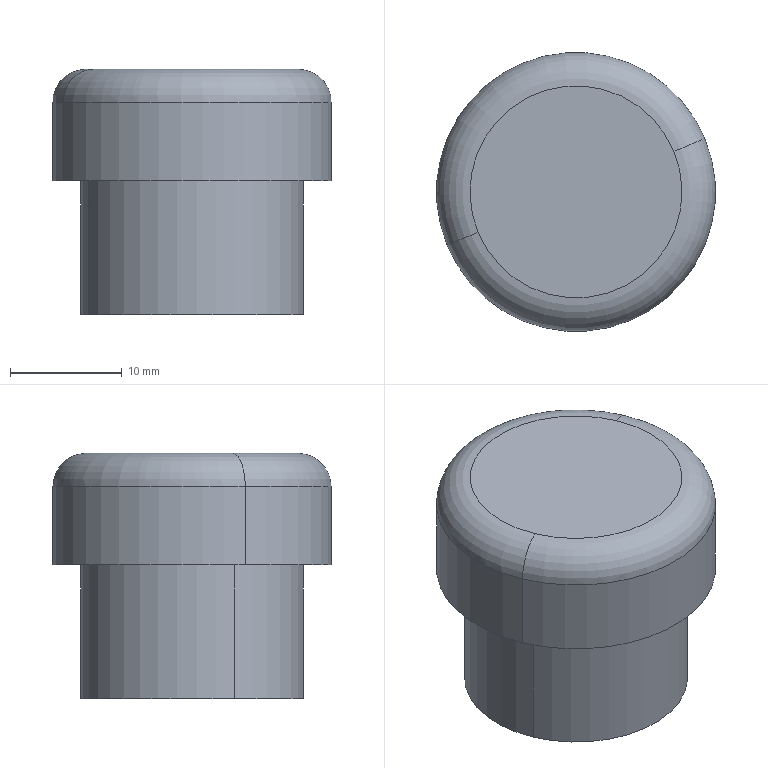Component | SolidWorks | DoubleFilmTransport-1_RubberPad-1 | 1 solid | 9 faces | box 25 x 25 x 22 mm | volume 8535 mm3 | cylinder 4 | plane 3 | torus 2 | commonest cylinder face diameters 25 x2 20 x2
build123d program:
from build123d import *


with BuildPart() as part:
    # Sketch1 → Revolve1 (revolve)
    with BuildSketch(Plane(origin=(0, 0, 0), x_dir=(-1, 0, 0), z_dir=(0, 0, -1)), mode=Mode.PRIVATE) as revolve1_sk:
        with BuildLine():
            Line((0, 10), (0, 0))
            Line((0, 0), (22, 0))
            Line((22, 0), (22, 9.5))
            ThreePointArc((22, 9.5), (21.121, 11.621), (19, 12.5))
            Line((19, 12.5), (12, 12.5))
            Line((12, 12.5), (12, 10))
            Line((12, 10), (0, 10))
        make_face()
    revolve(revolve1_sk.sketch.rotate(Axis((0, 0, 0), (-1, 0, 0)), 180), axis=Axis((0, 0, 0), (-1, 0, 0)))


solid = part.part

# Placed as in the assembly
solid = solid.moved(Location((-298.746, 95.373, 58.5), (0, 90, 0)))
STEP:
#1=CARTESIAN_POINT('',(-11.307,3.943,2.776));
#2=VERTEX_POINT('',#1);
#3=CARTESIAN_POINT('',(-12.217,3.567,2.776));
#4=VERTEX_POINT('',#3);
#5=CARTESIAN_POINT('',(-11.762,3.755,2.776));
#6=DIRECTION('',(0.,0.,1.));
#7=DIRECTION('',(0.9242,0.3818,0.));
#8=AXIS2_PLACEMENT_3D('',#5,#6,#7);
#9=CIRCLE('',#8,0.4921);
#10=EDGE_CURVE('',#2,#4,#9,.T.);
#11=ORIENTED_EDGE('',*,*,#10,.T.);
#12=CARTESIAN_POINT('',(-12.217,3.567,3.051));
#13=VERTEX_POINT('',#12);
#14=CARTESIAN_POINT('',(-12.217,3.567,2.303));
#15=DIRECTION('',(0.,0.,1.));
#16=VECTOR('',#15,39.37);
#17=LINE('',#14,#16);
#18=EDGE_CURVE('',#4,#13,#17,.T.);
#19=ORIENTED_EDGE('',*,*,#18,.T.);
#20=CARTESIAN_POINT('',(-11.307,3.943,3.051));
#21=VERTEX_POINT('',#20);
#22=CARTESIAN_POINT('',(-11.762,3.755,3.051));
#23=DIRECTION('',(0.,0.,1.));
#24=DIRECTION('',(0.9242,0.3818,0.));
#25=AXIS2_PLACEMENT_3D('',#22,#23,#24);
#26=CIRCLE('',#25,0.4921);
#27=EDGE_CURVE('',#21,#13,#26,.T.);
#28=ORIENTED_EDGE('',*,*,#27,.F.);
#29=CARTESIAN_POINT('',(-11.307,3.943,2.303));
#30=DIRECTION('',(0.,0.,1.));
#31=VECTOR('',#30,39.37);
#32=LINE('',#29,#31);
#33=EDGE_CURVE('',#2,#21,#32,.T.);
#34=ORIENTED_EDGE('',*,*,#33,.F.);
#35=EDGE_LOOP('',(#11,#19,#28,#34));
#36=FACE_OUTER_BOUND('',#35,.T.);
#37=CARTESIAN_POINT('',(-11.762,3.755,2.303));
#38=DIRECTION('',(0.,0.,1.));
#39=DIRECTION('',(0.9242,0.3818,0.));
#40=AXIS2_PLACEMENT_3D('',#37,#38,#39);
#41=CYLINDRICAL_SURFACE('',#40,0.4921);
#42=ADVANCED_FACE('',(#36),#41,.T.);
#43=ORIENTED_EDGE('',*,*,#27,.T.);
#44=CARTESIAN_POINT('',(-12.107,3.612,3.169));
#45=VERTEX_POINT('',#44);
#46=CARTESIAN_POINT('',(-12.107,3.612,3.051));
#47=DIRECTION('',(-0.3818,0.9242,0.));
#48=DIRECTION('',(-0.9242,-0.3818,0.));
#49=AXIS2_PLACEMENT_3D('',#46,#47,#48);
#50=CIRCLE('',#49,0.1181);
#51=EDGE_CURVE('',#13,#45,#50,.T.);
#52=ORIENTED_EDGE('',*,*,#51,.T.);
#53=CARTESIAN_POINT('',(-11.416,3.898,3.169));
#54=VERTEX_POINT('',#53);
#55=CARTESIAN_POINT('',(-11.762,3.755,3.169));
#56=DIRECTION('',(0.,0.,1.));
#57=DIRECTION('',(0.9242,0.3818,0.));
#58=AXIS2_PLACEMENT_3D('',#55,#56,#57);
#59=CIRCLE('',#58,0.374);
#60=EDGE_CURVE('',#54,#45,#59,.T.);
#61=ORIENTED_EDGE('',*,*,#60,.F.);
#62=CARTESIAN_POINT('',(-11.416,3.898,3.051));
#63=DIRECTION('',(0.3818,-0.9242,-0.));
#64=DIRECTION('',(0.9242,0.3818,0.));
#65=AXIS2_PLACEMENT_3D('',#62,#63,#64);
#66=CIRCLE('',#65,0.1181);
#67=EDGE_CURVE('',#21,#54,#66,.T.);
#68=ORIENTED_EDGE('',*,*,#67,.F.);
#69=EDGE_LOOP('',(#43,#52,#61,#68));
#70=FACE_OUTER_BOUND('',#69,.T.);
#71=CARTESIAN_POINT('',(-11.762,3.755,3.051));
#72=DIRECTION('',(0.,0.,1.));
#73=DIRECTION('',(0.9242,0.3818,-0.));
#74=AXIS2_PLACEMENT_3D('',#71,#72,#73);
#75=TOROIDAL_SURFACE('',#74,0.374,0.1181);
#76=ADVANCED_FACE('',(#70),#75,.T.);
#77=CARTESIAN_POINT('',(-11.398,3.905,2.303));
#78=VERTEX_POINT('',#77);
#79=CARTESIAN_POINT('',(-12.126,3.605,2.303));
#80=VERTEX_POINT('',#79);
#81=CARTESIAN_POINT('',(-11.762,3.755,2.303));
#82=DIRECTION('',(0.,0.,1.));
#83=DIRECTION('',(0.9242,0.3818,0.));
#84=AXIS2_PLACEMENT_3D('',#81,#82,#83);
#85=CIRCLE('',#84,0.3937);
#86=EDGE_CURVE('',#78,#80,#85,.T.);
#87=ORIENTED_EDGE('',*,*,#86,.T.);
#88=CARTESIAN_POINT('',(-12.126,3.605,2.776));
#89=VERTEX_POINT('',#88);
#90=CARTESIAN_POINT('',(-12.126,3.605,2.303));
#91=DIRECTION('',(0.,0.,1.));
#92=VECTOR('',#91,39.37);
#93=LINE('',#90,#92);
#94=EDGE_CURVE('',#80,#89,#93,.T.);
#95=ORIENTED_EDGE('',*,*,#94,.T.);
#96=CARTESIAN_POINT('',(-11.398,3.905,2.776));
#97=VERTEX_POINT('',#96);
#98=CARTESIAN_POINT('',(-11.762,3.755,2.776));
#99=DIRECTION('',(0.,0.,1.));
#100=DIRECTION('',(0.9242,0.3818,0.));
#101=AXIS2_PLACEMENT_3D('',#98,#99,#100);
#102=CIRCLE('',#101,0.3937);
#103=EDGE_CURVE('',#97,#89,#102,.T.);
#104=ORIENTED_EDGE('',*,*,#103,.F.);
#105=CARTESIAN_POINT('',(-11.398,3.905,2.303));
#106=DIRECTION('',(0.,0.,1.));
#107=VECTOR('',#106,39.37);
#108=LINE('',#105,#107);
#109=EDGE_CURVE('',#78,#97,#108,.T.);
#110=ORIENTED_EDGE('',*,*,#109,.F.);
#111=EDGE_LOOP('',(#87,#95,#104,#110));
#112=FACE_OUTER_BOUND('',#111,.T.);
#113=CARTESIAN_POINT('',(-11.762,3.755,2.303));
#114=DIRECTION('',(0.,0.,1.));
#115=DIRECTION('',(0.9242,0.3818,0.));
#116=AXIS2_PLACEMENT_3D('',#113,#114,#115);
#117=CYLINDRICAL_SURFACE('',#116,0.3937);
#118=ADVANCED_FACE('',(#112),#117,.T.);
#119=ORIENTED_EDGE('',*,*,#94,.F.);
#120=CARTESIAN_POINT('',(-11.762,3.755,2.303));
#121=DIRECTION('',(0.,0.,1.));
#122=DIRECTION('',(0.9242,0.3818,0.));
#123=AXIS2_PLACEMENT_3D('',#120,#121,#122);
#124=CIRCLE('',#123,0.3937);
#125=EDGE_CURVE('',#80,#78,#124,.T.);
#126=ORIENTED_EDGE('',*,*,#125,.T.);
#127=ORIENTED_EDGE('',*,*,#109,.T.);
#128=CARTESIAN_POINT('',(-11.762,3.755,2.776));
#129=DIRECTION('',(0.,0.,1.));
#130=DIRECTION('',(0.9242,0.3818,0.));
#131=AXIS2_PLACEMENT_3D('',#128,#129,#130);
#132=CIRCLE('',#131,0.3937);
#133=EDGE_CURVE('',#89,#97,#132,.T.);
#134=ORIENTED_EDGE('',*,*,#133,.F.);
#135=EDGE_LOOP('',(#119,#126,#127,#134));
#136=FACE_OUTER_BOUND('',#135,.T.);
#137=CARTESIAN_POINT('',(-11.762,3.755,2.303));
#138=DIRECTION('',(0.,0.,1.));
#139=DIRECTION('',(0.9242,0.3818,0.));
#140=AXIS2_PLACEMENT_3D('',#137,#138,#139);
#141=CYLINDRICAL_SURFACE('',#140,0.3937);
#142=ADVANCED_FACE('',(#136),#141,.T.);
#143=ORIENTED_EDGE('',*,*,#86,.F.);
#144=ORIENTED_EDGE('',*,*,#125,.F.);
#145=EDGE_LOOP('',(#143,#144));
#146=FACE_OUTER_BOUND('',#145,.T.);
#147=CARTESIAN_POINT('',(-12.126,3.605,2.303));
#148=DIRECTION('',(-0.,-0.,-1.));
#149=DIRECTION('',(-0.9242,-0.3818,0.));
#150=AXIS2_PLACEMENT_3D('',#147,#148,#149);
#151=PLANE('',#150);
#152=ADVANCED_FACE('',(#146),#151,.T.);
#153=ORIENTED_EDGE('',*,*,#60,.T.);
#154=CARTESIAN_POINT('',(-11.762,3.755,3.169));
#155=DIRECTION('',(0.,0.,1.));
#156=DIRECTION('',(0.9242,0.3818,0.));
#157=AXIS2_PLACEMENT_3D('',#154,#155,#156);
#158=CIRCLE('',#157,0.374);
#159=EDGE_CURVE('',#45,#54,#158,.T.);
#160=ORIENTED_EDGE('',*,*,#159,.T.);
#161=EDGE_LOOP('',(#153,#160));
#162=FACE_OUTER_BOUND('',#161,.T.);
#163=CARTESIAN_POINT('',(-11.762,3.755,3.169));
#164=DIRECTION('',(0.,0.,1.));
#165=DIRECTION('',(0.9242,0.3818,-0.));
#166=AXIS2_PLACEMENT_3D('',#163,#164,#165);
#167=PLANE('',#166);
#168=ADVANCED_FACE('',(#162),#167,.T.);
#169=ORIENTED_EDGE('',*,*,#51,.F.);
#170=CARTESIAN_POINT('',(-11.762,3.755,3.051));
#171=DIRECTION('',(0.,0.,1.));
#172=DIRECTION('',(0.9242,0.3818,0.));
#173=AXIS2_PLACEMENT_3D('',#170,#171,#172);
#174=CIRCLE('',#173,0.4921);
#175=EDGE_CURVE('',#13,#21,#174,.T.);
#176=ORIENTED_EDGE('',*,*,#175,.T.);
#177=ORIENTED_EDGE('',*,*,#67,.T.);
#178=ORIENTED_EDGE('',*,*,#159,.F.);
#179=EDGE_LOOP('',(#169,#176,#177,#178));
#180=FACE_OUTER_BOUND('',#179,.T.);
#181=CARTESIAN_POINT('',(-11.762,3.755,3.051));
#182=DIRECTION('',(0.,0.,1.));
#183=DIRECTION('',(0.9242,0.3818,-0.));
#184=AXIS2_PLACEMENT_3D('',#181,#182,#183);
#185=TOROIDAL_SURFACE('',#184,0.374,0.1181);
#186=ADVANCED_FACE('',(#180),#185,.T.);
#187=ORIENTED_EDGE('',*,*,#18,.F.);
#188=CARTESIAN_POINT('',(-11.762,3.755,2.776));
#189=DIRECTION('',(0.,0.,1.));
#190=DIRECTION('',(0.9242,0.3818,0.));
#191=AXIS2_PLACEMENT_3D('',#188,#189,#190);
#192=CIRCLE('',#191,0.4921);
#193=EDGE_CURVE('',#4,#2,#192,.T.);
#194=ORIENTED_EDGE('',*,*,#193,.T.);
#195=ORIENTED_EDGE('',*,*,#33,.T.);
#196=ORIENTED_EDGE('',*,*,#175,.F.);
#197=EDGE_LOOP('',(#187,#194,#195,#196));
#198=FACE_OUTER_BOUND('',#197,.T.);
#199=CARTESIAN_POINT('',(-11.762,3.755,2.303));
#200=DIRECTION('',(0.,0.,1.));
#201=DIRECTION('',(0.9242,0.3818,0.));
#202=AXIS2_PLACEMENT_3D('',#199,#200,#201);
#203=CYLINDRICAL_SURFACE('',#202,0.4921);
#204=ADVANCED_FACE('',(#198),#203,.T.);
#205=ORIENTED_EDGE('',*,*,#103,.T.);
#206=ORIENTED_EDGE('',*,*,#133,.T.);
#207=EDGE_LOOP('',(#205,#206));
#208=FACE_BOUND('',#207,.T.);
#209=ORIENTED_EDGE('',*,*,#10,.F.);
#210=ORIENTED_EDGE('',*,*,#193,.F.);
#211=EDGE_LOOP('',(#209,#210));
#212=FACE_OUTER_BOUND('',#211,.T.);
#213=CARTESIAN_POINT('',(-12.217,3.567,2.776));
#214=DIRECTION('',(-0.,-0.,-1.));
#215=DIRECTION('',(-0.9242,-0.3818,0.));
#216=AXIS2_PLACEMENT_3D('',#213,#214,#215);
#217=PLANE('',#216);
#218=ADVANCED_FACE('',(#208,#212),#217,.T.);
#219=CLOSED_SHELL('',(#42,#76,#118,#142,#152,#168,#186,#204,#218));
#220=MANIFOLD_SOLID_BREP('',#219);
#221=CARTESIAN_POINT('',(0.,0.,0.));
#222=DIRECTION('',(0.,0.,1.));
#223=DIRECTION('',(1.,0.,0.));
#224=AXIS2_PLACEMENT_3D('',#221,#222,#223);
#225=(LENGTH_UNIT()NAMED_UNIT(*)SI_UNIT($,.METRE.));
#226=LENGTH_MEASURE_WITH_UNIT(LENGTH_MEASURE(0.0254),#225);
#227=DIMENSIONAL_EXPONENTS(1.,0.,0.,0.,0.,0.,0.);
#228=(CONVERSION_BASED_UNIT('',#226)LENGTH_UNIT()NAMED_UNIT(#227));
#229=UNCERTAINTY_MEASURE_WITH_UNIT(LENGTH_MEASURE(0.00001),#228,'','');
#230=(NAMED_UNIT(*)PLANE_ANGLE_UNIT()SI_UNIT($,.RADIAN.));
#231=(NAMED_UNIT(*)SI_UNIT($,.STERADIAN.)SOLID_ANGLE_UNIT());
#232=(GEOMETRIC_REPRESENTATION_CONTEXT(3)GLOBAL_UNCERTAINTY_ASSIGNED_CONTEXT((#229))GLOBAL_UNIT_ASSIGNED_CONTEXT((#228,#230,#231))REPRESENTATION_CONTEXT('',''));
#233=ADVANCED_BREP_SHAPE_REPRESENTATION('',(#220,#224),#232);
#234=COLOUR_RGB('',0.7922,0.8196,0.9333);
#235=FILL_AREA_STYLE_COLOUR('',#234);
#236=FILL_AREA_STYLE('',(#235));
#237=SURFACE_STYLE_FILL_AREA(#236);
#238=SURFACE_SIDE_STYLE('',(#237));
#239=SURFACE_STYLE_USAGE(.BOTH.,#238);
#240=PRESENTATION_STYLE_ASSIGNMENT((#239));
#241=STYLED_ITEM('',(#240),#220);
#242=(LENGTH_UNIT()NAMED_UNIT(*)SI_UNIT($,.METRE.));
#243=LENGTH_MEASURE_WITH_UNIT(LENGTH_MEASURE(0.0254),#242);
#244=DIMENSIONAL_EXPONENTS(1.,0.,0.,0.,0.,0.,0.);
#245=(CONVERSION_BASED_UNIT('',#243)LENGTH_UNIT()NAMED_UNIT(#244));
#246=UNCERTAINTY_MEASURE_WITH_UNIT(LENGTH_MEASURE(0.00001),#245,'','');
#247=(NAMED_UNIT(*)PLANE_ANGLE_UNIT()SI_UNIT($,.RADIAN.));
#248=(NAMED_UNIT(*)SI_UNIT($,.STERADIAN.)SOLID_ANGLE_UNIT());
#249=(GEOMETRIC_REPRESENTATION_CONTEXT(3)GLOBAL_UNCERTAINTY_ASSIGNED_CONTEXT((#246))GLOBAL_UNIT_ASSIGNED_CONTEXT((#245,#247,#248))REPRESENTATION_CONTEXT('',''));
#250=MECHANICAL_DESIGN_GEOMETRIC_PRESENTATION_REPRESENTATION('',(#241),#249);
#251=PRESENTATION_LAYER_ASSIGNMENT('','',(#241));